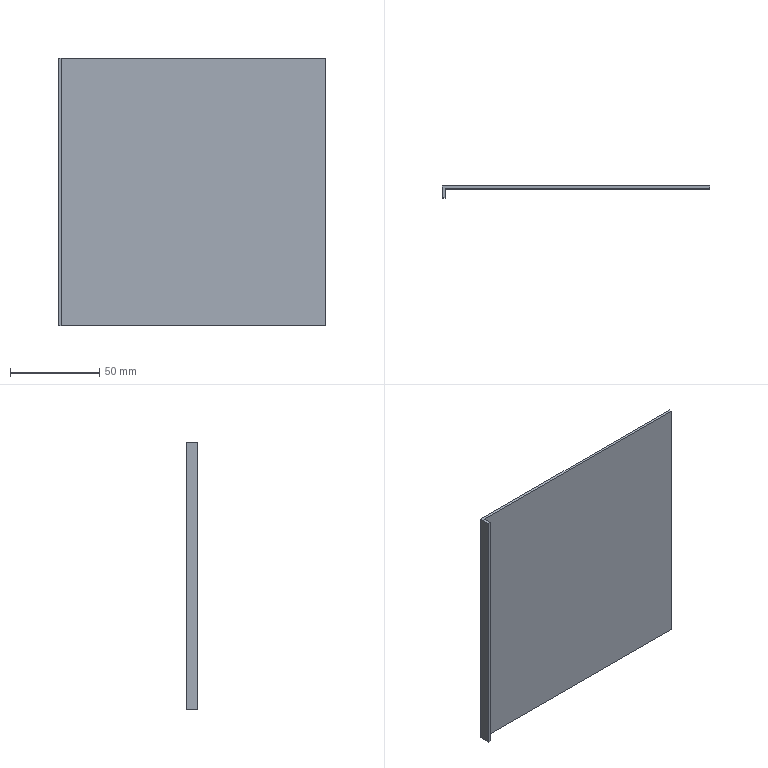Component | SolidWorks | LeftPlatform-1 | 1 solid | 8 faces | box 150 x 6.5 x 150 mm | volume 34875 mm3 | plane 8
build123d program:
from build123d import *

# Parameters (mm, degrees)
SKETCH1_W           = 150
SKETCH1_H           = 150
BOSS_EXTRUDE1_DEPTH = 1.5
SKETCH2_W           = 150
SKETCH2_H           = 6.5
BOSS_EXTRUDE2_DEPTH = 1.5


with BuildPart() as part:
    # Sketch1 → Boss-Extrude1 (new body)
    with BuildSketch(Plane(origin=(0, 0, 0), x_dir=(1, 0, 0), z_dir=(0, 1, 0))):
        Rectangle(SKETCH1_W, SKETCH1_H)
    extrude(amount=BOSS_EXTRUDE1_DEPTH)

    # Sketch2 → Boss-Extrude2 (add)
    with BuildSketch(Plane.ZY.offset(75)):
        with Locations((0, -1.75)):
            Rectangle(SKETCH2_W, SKETCH2_H)
    extrude(amount=-BOSS_EXTRUDE2_DEPTH)


solid = part.part

# Placed as in the assembly
solid = solid.moved(Location((-223.5, 597, 0), (0, 0, 0)))
STEP:
#1=COLOUR_RGB('',0.7922,0.8196,0.9333);
#2=FILL_AREA_STYLE_COLOUR('',#1);
#3=FILL_AREA_STYLE('',(#2));
#4=SURFACE_STYLE_FILL_AREA(#3);
#5=SURFACE_SIDE_STYLE('',(#4));
#6=SURFACE_STYLE_USAGE(.BOTH.,#5);
#7=PRESENTATION_STYLE_ASSIGNMENT((#6));
#8=CARTESIAN_POINT('',(-11.693,23.504,-2.953));
#9=VERTEX_POINT('',#8);
#10=CARTESIAN_POINT('',(-11.693,23.504,2.953));
#11=VERTEX_POINT('',#10);
#12=CARTESIAN_POINT('',(-11.693,23.504,0.));
#13=DIRECTION('',(0.,0.,1.));
#14=VECTOR('',#13,39.37);
#15=LINE('',#12,#14);
#16=EDGE_CURVE('',#9,#11,#15,.T.);
#17=ORIENTED_EDGE('',*,*,#16,.F.);
#18=CARTESIAN_POINT('',(-5.846,23.504,-2.953));
#19=VERTEX_POINT('',#18);
#20=CARTESIAN_POINT('',(-11.752,23.504,-2.953));
#21=DIRECTION('',(-1.,0.,0.));
#22=VECTOR('',#21,39.37);
#23=LINE('',#20,#22);
#24=EDGE_CURVE('',#19,#9,#23,.T.);
#25=ORIENTED_EDGE('',*,*,#24,.F.);
#26=CARTESIAN_POINT('',(-5.846,23.504,2.953));
#27=VERTEX_POINT('',#26);
#28=CARTESIAN_POINT('',(-5.846,23.504,-2.953));
#29=DIRECTION('',(0.,0.,-1.));
#30=VECTOR('',#29,39.37);
#31=LINE('',#28,#30);
#32=EDGE_CURVE('',#27,#19,#31,.T.);
#33=ORIENTED_EDGE('',*,*,#32,.F.);
#34=CARTESIAN_POINT('',(-11.752,23.504,2.953));
#35=DIRECTION('',(1.,0.,0.));
#36=VECTOR('',#35,39.37);
#37=LINE('',#34,#36);
#38=EDGE_CURVE('',#11,#27,#37,.T.);
#39=ORIENTED_EDGE('',*,*,#38,.F.);
#40=EDGE_LOOP('',(#17,#25,#33,#39));
#41=FACE_OUTER_BOUND('',#40,.T.);
#42=CARTESIAN_POINT('',(-8.799,23.504,0.));
#43=DIRECTION('',(0.,1.,0.));
#44=DIRECTION('',(0.,0.,1.));
#45=AXIS2_PLACEMENT_3D('',#42,#43,#44);
#46=PLANE('',#45);
#47=ADVANCED_FACE('',(#41),#46,.F.);
#48=ORIENTED_EDGE('',*,*,#32,.T.);
#49=CARTESIAN_POINT('',(-5.846,23.563,-2.953));
#50=VERTEX_POINT('',#49);
#51=CARTESIAN_POINT('',(-5.846,23.563,-2.953));
#52=DIRECTION('',(0.,-1.,0.));
#53=VECTOR('',#52,39.37);
#54=LINE('',#51,#53);
#55=EDGE_CURVE('',#50,#19,#54,.T.);
#56=ORIENTED_EDGE('',*,*,#55,.F.);
#57=CARTESIAN_POINT('',(-5.846,23.563,2.953));
#58=VERTEX_POINT('',#57);
#59=CARTESIAN_POINT('',(-5.846,23.563,-2.953));
#60=DIRECTION('',(0.,0.,-1.));
#61=VECTOR('',#60,39.37);
#62=LINE('',#59,#61);
#63=EDGE_CURVE('',#58,#50,#62,.T.);
#64=ORIENTED_EDGE('',*,*,#63,.F.);
#65=CARTESIAN_POINT('',(-5.846,23.563,2.953));
#66=DIRECTION('',(0.,-1.,0.));
#67=VECTOR('',#66,39.37);
#68=LINE('',#65,#67);
#69=EDGE_CURVE('',#58,#27,#68,.T.);
#70=ORIENTED_EDGE('',*,*,#69,.T.);
#71=EDGE_LOOP('',(#48,#56,#64,#70));
#72=FACE_OUTER_BOUND('',#71,.T.);
#73=CARTESIAN_POINT('',(-5.846,23.563,-2.953));
#74=DIRECTION('',(-1.,0.,0.));
#75=DIRECTION('',(0.,0.,1.));
#76=AXIS2_PLACEMENT_3D('',#73,#74,#75);
#77=PLANE('',#76);
#78=ADVANCED_FACE('',(#72),#77,.F.);
#79=CARTESIAN_POINT('',(-11.752,23.563,-2.953));
#80=VERTEX_POINT('',#79);
#81=CARTESIAN_POINT('',(-11.752,23.307,-2.953));
#82=VERTEX_POINT('',#81);
#83=CARTESIAN_POINT('',(-11.752,23.563,-2.953));
#84=DIRECTION('',(0.,-1.,0.));
#85=VECTOR('',#84,39.37);
#86=LINE('',#83,#85);
#87=EDGE_CURVE('',#80,#82,#86,.T.);
#88=ORIENTED_EDGE('',*,*,#87,.F.);
#89=CARTESIAN_POINT('',(-11.752,23.563,-2.953));
#90=DIRECTION('',(-1.,0.,0.));
#91=VECTOR('',#90,39.37);
#92=LINE('',#89,#91);
#93=EDGE_CURVE('',#50,#80,#92,.T.);
#94=ORIENTED_EDGE('',*,*,#93,.F.);
#95=ORIENTED_EDGE('',*,*,#55,.T.);
#96=ORIENTED_EDGE('',*,*,#24,.T.);
#97=CARTESIAN_POINT('',(-11.693,23.307,-2.953));
#98=VERTEX_POINT('',#97);
#99=CARTESIAN_POINT('',(-11.693,23.563,-2.953));
#100=DIRECTION('',(0.,-1.,0.));
#101=VECTOR('',#100,39.37);
#102=LINE('',#99,#101);
#103=EDGE_CURVE('',#9,#98,#102,.T.);
#104=ORIENTED_EDGE('',*,*,#103,.T.);
#105=CARTESIAN_POINT('',(-11.693,23.307,-2.953));
#106=DIRECTION('',(-1.,0.,0.));
#107=VECTOR('',#106,39.37);
#108=LINE('',#105,#107);
#109=EDGE_CURVE('',#98,#82,#108,.T.);
#110=ORIENTED_EDGE('',*,*,#109,.T.);
#111=EDGE_LOOP('',(#88,#94,#95,#96,#104,#110));
#112=FACE_OUTER_BOUND('',#111,.T.);
#113=CARTESIAN_POINT('',(-11.752,23.563,-2.953));
#114=DIRECTION('',(0.,0.,1.));
#115=DIRECTION('',(1.,0.,0.));
#116=AXIS2_PLACEMENT_3D('',#113,#114,#115);
#117=PLANE('',#116);
#118=ADVANCED_FACE('',(#112),#117,.F.);
#119=ORIENTED_EDGE('',*,*,#87,.T.);
#120=CARTESIAN_POINT('',(-11.752,23.307,2.953));
#121=VERTEX_POINT('',#120);
#122=CARTESIAN_POINT('',(-11.752,23.307,-2.953));
#123=DIRECTION('',(0.,0.,1.));
#124=VECTOR('',#123,39.37);
#125=LINE('',#122,#124);
#126=EDGE_CURVE('',#82,#121,#125,.T.);
#127=ORIENTED_EDGE('',*,*,#126,.T.);
#128=CARTESIAN_POINT('',(-11.752,23.563,2.953));
#129=VERTEX_POINT('',#128);
#130=CARTESIAN_POINT('',(-11.752,23.563,2.953));
#131=DIRECTION('',(0.,-1.,0.));
#132=VECTOR('',#131,39.37);
#133=LINE('',#130,#132);
#134=EDGE_CURVE('',#129,#121,#133,.T.);
#135=ORIENTED_EDGE('',*,*,#134,.F.);
#136=CARTESIAN_POINT('',(-11.752,23.563,-2.953));
#137=DIRECTION('',(0.,0.,1.));
#138=VECTOR('',#137,39.37);
#139=LINE('',#136,#138);
#140=EDGE_CURVE('',#80,#129,#139,.T.);
#141=ORIENTED_EDGE('',*,*,#140,.F.);
#142=EDGE_LOOP('',(#119,#127,#135,#141));
#143=FACE_OUTER_BOUND('',#142,.T.);
#144=CARTESIAN_POINT('',(-11.752,23.563,-2.953));
#145=DIRECTION('',(1.,0.,0.));
#146=DIRECTION('',(0.,0.,-1.));
#147=AXIS2_PLACEMENT_3D('',#144,#145,#146);
#148=PLANE('',#147);
#149=ADVANCED_FACE('',(#143),#148,.F.);
#150=ORIENTED_EDGE('',*,*,#134,.T.);
#151=CARTESIAN_POINT('',(-11.693,23.307,2.953));
#152=VERTEX_POINT('',#151);
#153=CARTESIAN_POINT('',(-11.693,23.307,2.953));
#154=DIRECTION('',(-1.,0.,0.));
#155=VECTOR('',#154,39.37);
#156=LINE('',#153,#155);
#157=EDGE_CURVE('',#152,#121,#156,.T.);
#158=ORIENTED_EDGE('',*,*,#157,.F.);
#159=CARTESIAN_POINT('',(-11.693,23.563,2.953));
#160=DIRECTION('',(0.,1.,0.));
#161=VECTOR('',#160,39.37);
#162=LINE('',#159,#161);
#163=EDGE_CURVE('',#152,#11,#162,.T.);
#164=ORIENTED_EDGE('',*,*,#163,.T.);
#165=ORIENTED_EDGE('',*,*,#38,.T.);
#166=ORIENTED_EDGE('',*,*,#69,.F.);
#167=CARTESIAN_POINT('',(-11.752,23.563,2.953));
#168=DIRECTION('',(1.,0.,0.));
#169=VECTOR('',#168,39.37);
#170=LINE('',#167,#169);
#171=EDGE_CURVE('',#129,#58,#170,.T.);
#172=ORIENTED_EDGE('',*,*,#171,.F.);
#173=EDGE_LOOP('',(#150,#158,#164,#165,#166,#172));
#174=FACE_OUTER_BOUND('',#173,.T.);
#175=CARTESIAN_POINT('',(-11.752,23.563,2.953));
#176=DIRECTION('',(0.,0.,-1.));
#177=DIRECTION('',(-1.,0.,0.));
#178=AXIS2_PLACEMENT_3D('',#175,#176,#177);
#179=PLANE('',#178);
#180=ADVANCED_FACE('',(#174),#179,.F.);
#181=ORIENTED_EDGE('',*,*,#171,.T.);
#182=ORIENTED_EDGE('',*,*,#63,.T.);
#183=ORIENTED_EDGE('',*,*,#93,.T.);
#184=ORIENTED_EDGE('',*,*,#140,.T.);
#185=EDGE_LOOP('',(#181,#182,#183,#184));
#186=FACE_OUTER_BOUND('',#185,.T.);
#187=CARTESIAN_POINT('',(-8.799,23.563,0.));
#188=DIRECTION('',(0.,1.,0.));
#189=DIRECTION('',(0.,0.,1.));
#190=AXIS2_PLACEMENT_3D('',#187,#188,#189);
#191=PLANE('',#190);
#192=ADVANCED_FACE('',(#186),#191,.T.);
#193=ORIENTED_EDGE('',*,*,#103,.F.);
#194=ORIENTED_EDGE('',*,*,#16,.T.);
#195=ORIENTED_EDGE('',*,*,#163,.F.);
#196=CARTESIAN_POINT('',(-11.693,23.307,-2.953));
#197=DIRECTION('',(0.,0.,1.));
#198=VECTOR('',#197,39.37);
#199=LINE('',#196,#198);
#200=EDGE_CURVE('',#98,#152,#199,.T.);
#201=ORIENTED_EDGE('',*,*,#200,.F.);
#202=EDGE_LOOP('',(#193,#194,#195,#201));
#203=FACE_OUTER_BOUND('',#202,.T.);
#204=CARTESIAN_POINT('',(-11.693,23.504,0.));
#205=DIRECTION('',(-1.,0.,0.));
#206=DIRECTION('',(0.,0.,1.));
#207=AXIS2_PLACEMENT_3D('',#204,#205,#206);
#208=PLANE('',#207);
#209=ADVANCED_FACE('',(#203),#208,.F.);
#210=ORIENTED_EDGE('',*,*,#126,.F.);
#211=ORIENTED_EDGE('',*,*,#109,.F.);
#212=ORIENTED_EDGE('',*,*,#200,.T.);
#213=ORIENTED_EDGE('',*,*,#157,.T.);
#214=EDGE_LOOP('',(#210,#211,#212,#213));
#215=FACE_OUTER_BOUND('',#214,.T.);
#216=CARTESIAN_POINT('',(-11.693,23.307,-2.953));
#217=DIRECTION('',(0.,-1.,0.));
#218=DIRECTION('',(0.,0.,-1.));
#219=AXIS2_PLACEMENT_3D('',#216,#217,#218);
#220=PLANE('',#219);
#221=ADVANCED_FACE('',(#215),#220,.T.);
#222=CLOSED_SHELL('',(#47,#78,#118,#149,#180,#192,#209,#221));
#223=MANIFOLD_SOLID_BREP('',#222);
#224=STYLED_ITEM('',(#7),#223);
#225=PRESENTATION_LAYER_ASSIGNMENT('','',(#224));
#226=(LENGTH_UNIT()NAMED_UNIT(*)SI_UNIT($,.METRE.));
#227=LENGTH_MEASURE_WITH_UNIT(LENGTH_MEASURE(0.0254),#226);
#228=DIMENSIONAL_EXPONENTS(1.,0.,0.,0.,0.,0.,0.);
#229=(CONVERSION_BASED_UNIT('',#227)LENGTH_UNIT()NAMED_UNIT(#228));
#230=UNCERTAINTY_MEASURE_WITH_UNIT(LENGTH_MEASURE(0.00001),#229,'','');
#231=(NAMED_UNIT(*)PLANE_ANGLE_UNIT()SI_UNIT($,.RADIAN.));
#232=(NAMED_UNIT(*)SI_UNIT($,.STERADIAN.)SOLID_ANGLE_UNIT());
#233=(GEOMETRIC_REPRESENTATION_CONTEXT(3)GLOBAL_UNCERTAINTY_ASSIGNED_CONTEXT((#230))GLOBAL_UNIT_ASSIGNED_CONTEXT((#229,#231,#232))REPRESENTATION_CONTEXT('',''));
#234=MECHANICAL_DESIGN_GEOMETRIC_PRESENTATION_REPRESENTATION('',(#224),#233);
#235=CARTESIAN_POINT('',(0.,0.,0.));
#236=DIRECTION('',(0.,0.,1.));
#237=DIRECTION('',(1.,0.,0.));
#238=AXIS2_PLACEMENT_3D('',#235,#236,#237);
#239=(LENGTH_UNIT()NAMED_UNIT(*)SI_UNIT($,.METRE.));
#240=LENGTH_MEASURE_WITH_UNIT(LENGTH_MEASURE(0.0254),#239);
#241=DIMENSIONAL_EXPONENTS(1.,0.,0.,0.,0.,0.,0.);
#242=(CONVERSION_BASED_UNIT('',#240)LENGTH_UNIT()NAMED_UNIT(#241));
#243=UNCERTAINTY_MEASURE_WITH_UNIT(LENGTH_MEASURE(0.00001),#242,'','');
#244=(NAMED_UNIT(*)PLANE_ANGLE_UNIT()SI_UNIT($,.RADIAN.));
#245=(NAMED_UNIT(*)SI_UNIT($,.STERADIAN.)SOLID_ANGLE_UNIT());
#246=(GEOMETRIC_REPRESENTATION_CONTEXT(3)GLOBAL_UNCERTAINTY_ASSIGNED_CONTEXT((#243))GLOBAL_UNIT_ASSIGNED_CONTEXT((#242,#244,#245))REPRESENTATION_CONTEXT('',''));
#247=ADVANCED_BREP_SHAPE_REPRESENTATION('',(#223,#238),#246);